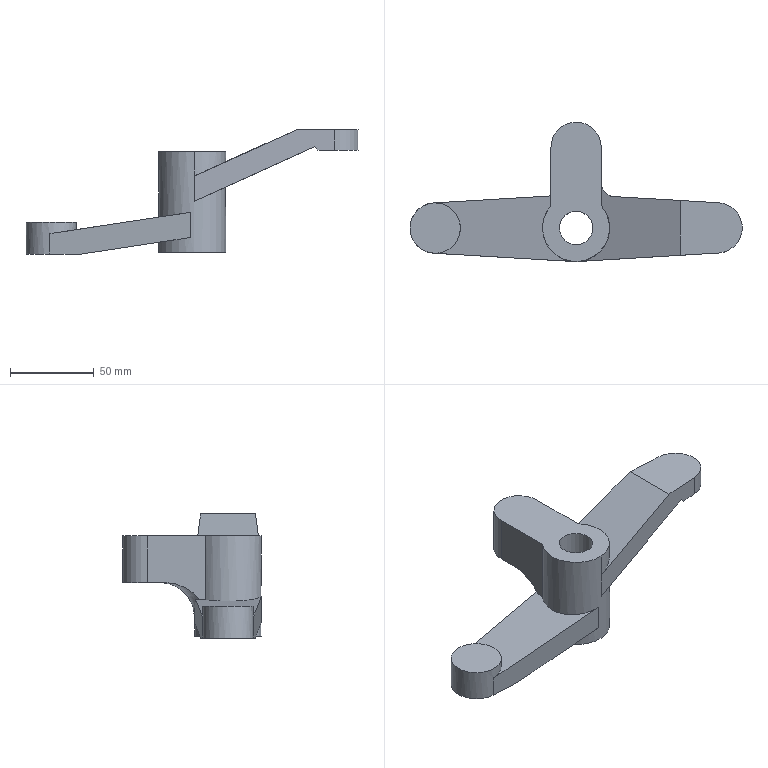Component | NX | EQUAL_ARM_LEVER_BLANK | 1 solid | 32 faces | volume 173754 mm3 | plane 23 | cylinder 8 | torus 1 | commonest cylinder face diameters 30 x3 40 x2 16 x1 8 x1 20 x1